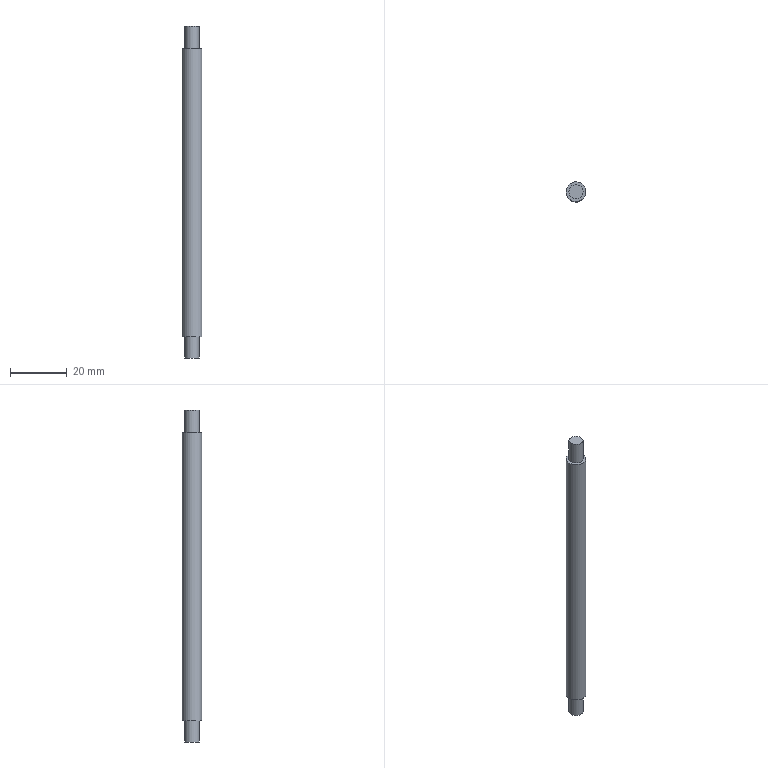Component | NX | COLUMN_4 | 1 solid | 7 faces | box 7 x 7 x 117.5 mm | volume 4230 mm3 | plane 4 | cylinder 3 | commonest cylinder face diameters 5 x2 7 x1
STEP:
#1=CARTESIAN_POINT('',(0.,0.,0.));
#2=DIRECTION('',(0.,0.,1.));
#3=DIRECTION('',(1.,0.,0.));
#4=AXIS2_PLACEMENT_3D('',#1,#2,#3);
#5=CARTESIAN_POINT('',(-21.585,4.647,11.));
#6=VERTEX_POINT('',#5);
#7=CARTESIAN_POINT('',(-24.,4.,11.));
#8=DIRECTION('',(0.,0.,1.));
#9=DIRECTION('',(0.9659,0.2588,0.));
#10=AXIS2_PLACEMENT_3D('',#7,#8,#9);
#11=CIRCLE('',#10,2.5);
#12=CARTESIAN_POINT('',(-24.,4.,11.));
#13=DIRECTION('',(0.,0.,-1.));
#14=DIRECTION('',(-0.9659,-0.2588,0.));
#15=AXIS2_PLACEMENT_3D('',#12,#13,#14);
#16=PLANE('',#15);
#17=CARTESIAN_POINT('',(-2.5,-0.));
#18=CARTESIAN_POINT('',(-2.5,4.33));
#19=CARTESIAN_POINT('',(1.25,2.165));
#20=CARTESIAN_POINT('',(5.,0.));
#21=CARTESIAN_POINT('',(1.25,-2.165));
#22=CARTESIAN_POINT('',(-2.5,-4.33));
#23=CARTESIAN_POINT('',(-2.5,-0.));
#24=(BOUNDED_CURVE()B_SPLINE_CURVE(2,(#17,#18,#19,#20,#21,#22,#23),.UNSPECIFIED.,.T.,.F.)B_SPLINE_CURVE_WITH_KNOTS((1,2,2,2,2,1),(-2.094,0.,2.094,4.189,6.283,8.378),.UNSPECIFIED.)CURVE()GEOMETRIC_REPRESENTATION_ITEM()RATIONAL_B_SPLINE_CURVE((1.,0.5,1.,0.5,1.,0.5,1.))REPRESENTATION_ITEM(''));
#25=(GEOMETRIC_REPRESENTATION_CONTEXT(2)PARAMETRIC_REPRESENTATION_CONTEXT()REPRESENTATION_CONTEXT('',''));
#26=DEFINITIONAL_REPRESENTATION('',(#24),#25);
#27=PCURVE('',#16,#26);
#28=CARTESIAN_POINT('',(-24.,4.,11.));
#29=DIRECTION('',(0.,0.,1.));
#30=DIRECTION('',(0.9659,0.2588,0.));
#31=AXIS2_PLACEMENT_3D('',#28,#29,#30);
#32=CYLINDRICAL_SURFACE('',#31,2.5);
#33=CARTESIAN_POINT('',(0.,0.));
#34=DIRECTION('',(1.,0.));
#35=VECTOR('',#34,1.);
#36=LINE('',#33,#35);
#37=(GEOMETRIC_REPRESENTATION_CONTEXT(2)PARAMETRIC_REPRESENTATION_CONTEXT()REPRESENTATION_CONTEXT('',''));
#38=DEFINITIONAL_REPRESENTATION('',(#36),#37);
#39=PCURVE('',#32,#38);
#40=SURFACE_CURVE('',#11,(#27,#39),.PCURVE_S1.);
#41=EDGE_CURVE('',#6,#6,#40,.T.);
#42=ORIENTED_EDGE('',*,*,#41,.F.);
#43=EDGE_LOOP('',(#42));
#44=FACE_BOUND('',#43,.T.);
#45=ADVANCED_FACE('',(#44),#16,.T.);
#46=CARTESIAN_POINT('',(-21.585,4.647,18.5));
#47=VERTEX_POINT('',#46);
#48=CARTESIAN_POINT('',(-24.,4.,18.5));
#49=DIRECTION('',(0.,0.,-1.));
#50=DIRECTION('',(0.9659,0.2588,0.));
#51=AXIS2_PLACEMENT_3D('',#48,#49,#50);
#52=CIRCLE('',#51,2.5);
#53=CARTESIAN_POINT('',(6.283,7.5));
#54=DIRECTION('',(-1.,0.));
#55=VECTOR('',#54,1.);
#56=LINE('',#53,#55);
#57=(GEOMETRIC_REPRESENTATION_CONTEXT(2)PARAMETRIC_REPRESENTATION_CONTEXT()REPRESENTATION_CONTEXT('',''));
#58=DEFINITIONAL_REPRESENTATION('',(#56),#57);
#59=PCURVE('',#32,#58);
#60=CARTESIAN_POINT('',(-24.,4.,18.5));
#61=DIRECTION('',(0.,0.,-1.));
#62=DIRECTION('',(-0.9659,-0.2588,0.));
#63=AXIS2_PLACEMENT_3D('',#60,#61,#62);
#64=PLANE('',#63);
#65=CARTESIAN_POINT('',(0.,0.));
#66=DIRECTION('',(-1.,-0.));
#67=AXIS2_PLACEMENT_2D('',#65,#66);
#68=CIRCLE('',#67,2.5);
#69=(GEOMETRIC_REPRESENTATION_CONTEXT(2)PARAMETRIC_REPRESENTATION_CONTEXT()REPRESENTATION_CONTEXT('',''));
#70=DEFINITIONAL_REPRESENTATION('',(#68),#69);
#71=PCURVE('',#64,#70);
#72=SURFACE_CURVE('',#52,(#59,#71),.PCURVE_S1.);
#73=EDGE_CURVE('',#47,#47,#72,.T.);
#74=ORIENTED_EDGE('',*,*,#73,.T.);
#75=CARTESIAN_POINT('',(-21.585,4.647,11.));
#76=CARTESIAN_POINT('',(-21.585,4.647,18.5));
#77=B_SPLINE_CURVE_WITH_KNOTS('',1,(#75,#76),.UNSPECIFIED.,.F.,.F.,(2,2),(0.,7.5),.PIECEWISE_BEZIER_KNOTS.);
#78=CARTESIAN_POINT('',(0.,0.));
#79=DIRECTION('',(0.,1.));
#80=VECTOR('',#79,1.);
#81=LINE('',#78,#80);
#82=(GEOMETRIC_REPRESENTATION_CONTEXT(2)PARAMETRIC_REPRESENTATION_CONTEXT()REPRESENTATION_CONTEXT('',''));
#83=DEFINITIONAL_REPRESENTATION('',(#81),#82);
#84=PCURVE('',#32,#83);
#85=CARTESIAN_POINT('',(6.283,0.));
#86=DIRECTION('',(0.,1.));
#87=VECTOR('',#86,1.);
#88=LINE('',#85,#87);
#89=(GEOMETRIC_REPRESENTATION_CONTEXT(2)PARAMETRIC_REPRESENTATION_CONTEXT()REPRESENTATION_CONTEXT('',''));
#90=DEFINITIONAL_REPRESENTATION('',(#88),#89);
#91=PCURVE('',#32,#90);
#92=SEAM_CURVE('',#77,(#84,#91),.PCURVE_S1.);
#93=EDGE_CURVE('',#6,#47,#92,.T.);
#94=ORIENTED_EDGE('',*,*,#93,.F.);
#95=ORIENTED_EDGE('',*,*,#41,.T.);
#96=ORIENTED_EDGE('',*,*,#93,.T.);
#97=EDGE_LOOP('',(#74,#94,#95,#96));
#98=FACE_BOUND('',#97,.T.);
#99=ADVANCED_FACE('',(#98),#32,.T.);
#100=CARTESIAN_POINT('',(-21.585,4.647,120.5));
#101=VERTEX_POINT('',#100);
#102=CARTESIAN_POINT('',(-24.,4.,120.5));
#103=DIRECTION('',(0.,0.,1.));
#104=DIRECTION('',(0.9659,0.2588,0.));
#105=AXIS2_PLACEMENT_3D('',#102,#103,#104);
#106=CIRCLE('',#105,2.5);
#107=CARTESIAN_POINT('',(-24.,4.,120.5));
#108=DIRECTION('',(0.,0.,1.));
#109=DIRECTION('',(0.9659,0.2588,0.));
#110=AXIS2_PLACEMENT_3D('',#107,#108,#109);
#111=PLANE('',#110);
#112=CARTESIAN_POINT('',(0.,0.));
#113=DIRECTION('',(1.,-0.));
#114=AXIS2_PLACEMENT_2D('',#112,#113);
#115=CIRCLE('',#114,2.5);
#116=(GEOMETRIC_REPRESENTATION_CONTEXT(2)PARAMETRIC_REPRESENTATION_CONTEXT()REPRESENTATION_CONTEXT('',''));
#117=DEFINITIONAL_REPRESENTATION('',(#115),#116);
#118=PCURVE('',#111,#117);
#119=CARTESIAN_POINT('',(-24.,4.,120.5));
#120=DIRECTION('',(0.,0.,1.));
#121=DIRECTION('',(0.9659,0.2588,0.));
#122=AXIS2_PLACEMENT_3D('',#119,#120,#121);
#123=CYLINDRICAL_SURFACE('',#122,2.5);
#124=CARTESIAN_POINT('',(0.,0.));
#125=DIRECTION('',(1.,0.));
#126=VECTOR('',#125,1.);
#127=LINE('',#124,#126);
#128=(GEOMETRIC_REPRESENTATION_CONTEXT(2)PARAMETRIC_REPRESENTATION_CONTEXT()REPRESENTATION_CONTEXT('',''));
#129=DEFINITIONAL_REPRESENTATION('',(#127),#128);
#130=PCURVE('',#123,#129);
#131=SURFACE_CURVE('',#106,(#118,#130),.PCURVE_S1.);
#132=EDGE_CURVE('',#101,#101,#131,.T.);
#133=ORIENTED_EDGE('',*,*,#132,.F.);
#134=EDGE_LOOP('',(#133));
#135=FACE_BOUND('',#134,.T.);
#136=CARTESIAN_POINT('',(-20.619,4.906,120.5));
#137=VERTEX_POINT('',#136);
#138=CARTESIAN_POINT('',(-24.,4.,120.5));
#139=DIRECTION('',(0.,0.,1.));
#140=DIRECTION('',(0.9659,0.2588,0.));
#141=AXIS2_PLACEMENT_3D('',#138,#139,#140);
#142=CIRCLE('',#141,3.5);
#143=CARTESIAN_POINT('',(0.,0.));
#144=DIRECTION('',(1.,0.));
#145=AXIS2_PLACEMENT_2D('',#143,#144);
#146=CIRCLE('',#145,3.5);
#147=(GEOMETRIC_REPRESENTATION_CONTEXT(2)PARAMETRIC_REPRESENTATION_CONTEXT()REPRESENTATION_CONTEXT('',''));
#148=DEFINITIONAL_REPRESENTATION('',(#146),#147);
#149=PCURVE('',#111,#148);
#150=CARTESIAN_POINT('',(-24.,4.,18.5));
#151=DIRECTION('',(0.,0.,1.));
#152=DIRECTION('',(0.9659,0.2588,0.));
#153=AXIS2_PLACEMENT_3D('',#150,#151,#152);
#154=CYLINDRICAL_SURFACE('',#153,3.5);
#155=CARTESIAN_POINT('',(0.,102.));
#156=DIRECTION('',(1.,0.));
#157=VECTOR('',#156,1.);
#158=LINE('',#155,#157);
#159=(GEOMETRIC_REPRESENTATION_CONTEXT(2)PARAMETRIC_REPRESENTATION_CONTEXT()REPRESENTATION_CONTEXT('',''));
#160=DEFINITIONAL_REPRESENTATION('',(#158),#159);
#161=PCURVE('',#154,#160);
#162=SURFACE_CURVE('',#142,(#149,#161),.PCURVE_S1.);
#163=EDGE_CURVE('',#137,#137,#162,.T.);
#164=ORIENTED_EDGE('',*,*,#163,.T.);
#165=EDGE_LOOP('',(#164));
#166=FACE_BOUND('',#165,.T.);
#167=ADVANCED_FACE('',(#135,#166),#111,.T.);
#168=ORIENTED_EDGE('',*,*,#73,.F.);
#169=EDGE_LOOP('',(#168));
#170=FACE_BOUND('',#169,.T.);
#171=CARTESIAN_POINT('',(-20.619,4.906,18.5));
#172=VERTEX_POINT('',#171);
#173=CARTESIAN_POINT('',(-24.,4.,18.5));
#174=DIRECTION('',(0.,0.,1.));
#175=DIRECTION('',(0.9659,0.2588,0.));
#176=AXIS2_PLACEMENT_3D('',#173,#174,#175);
#177=CIRCLE('',#176,3.5);
#178=CARTESIAN_POINT('',(-3.5,0.));
#179=CARTESIAN_POINT('',(-3.5,6.062));
#180=CARTESIAN_POINT('',(1.75,3.031));
#181=CARTESIAN_POINT('',(7.,0.));
#182=CARTESIAN_POINT('',(1.75,-3.031));
#183=CARTESIAN_POINT('',(-3.5,-6.062));
#184=CARTESIAN_POINT('',(-3.5,0.));
#185=(BOUNDED_CURVE()B_SPLINE_CURVE(2,(#178,#179,#180,#181,#182,#183,#184),.UNSPECIFIED.,.T.,.F.)B_SPLINE_CURVE_WITH_KNOTS((1,2,2,2,2,1),(-2.094,0.,2.094,4.189,6.283,8.378),.UNSPECIFIED.)CURVE()GEOMETRIC_REPRESENTATION_ITEM()RATIONAL_B_SPLINE_CURVE((1.,0.5,1.,0.5,1.,0.5,1.))REPRESENTATION_ITEM(''));
#186=(GEOMETRIC_REPRESENTATION_CONTEXT(2)PARAMETRIC_REPRESENTATION_CONTEXT()REPRESENTATION_CONTEXT('',''));
#187=DEFINITIONAL_REPRESENTATION('',(#185),#186);
#188=PCURVE('',#64,#187);
#189=CARTESIAN_POINT('',(0.,0.));
#190=DIRECTION('',(1.,0.));
#191=VECTOR('',#190,1.);
#192=LINE('',#189,#191);
#193=(GEOMETRIC_REPRESENTATION_CONTEXT(2)PARAMETRIC_REPRESENTATION_CONTEXT()REPRESENTATION_CONTEXT('',''));
#194=DEFINITIONAL_REPRESENTATION('',(#192),#193);
#195=PCURVE('',#154,#194);
#196=SURFACE_CURVE('',#177,(#188,#195),.PCURVE_S1.);
#197=EDGE_CURVE('',#172,#172,#196,.T.);
#198=ORIENTED_EDGE('',*,*,#197,.F.);
#199=EDGE_LOOP('',(#198));
#200=FACE_BOUND('',#199,.T.);
#201=ADVANCED_FACE('',(#170,#200),#64,.T.);
#202=ORIENTED_EDGE('',*,*,#163,.F.);
#203=CARTESIAN_POINT('',(-20.619,4.906,18.5));
#204=CARTESIAN_POINT('',(-20.619,4.906,120.5));
#205=B_SPLINE_CURVE_WITH_KNOTS('',1,(#203,#204),.UNSPECIFIED.,.F.,.F.,(2,2),(0.,102.),.PIECEWISE_BEZIER_KNOTS.);
#206=CARTESIAN_POINT('',(0.,0.));
#207=DIRECTION('',(0.,1.));
#208=VECTOR('',#207,1.);
#209=LINE('',#206,#208);
#210=(GEOMETRIC_REPRESENTATION_CONTEXT(2)PARAMETRIC_REPRESENTATION_CONTEXT()REPRESENTATION_CONTEXT('',''));
#211=DEFINITIONAL_REPRESENTATION('',(#209),#210);
#212=PCURVE('',#154,#211);
#213=CARTESIAN_POINT('',(6.283,0.));
#214=DIRECTION('',(0.,1.));
#215=VECTOR('',#214,1.);
#216=LINE('',#213,#215);
#217=(GEOMETRIC_REPRESENTATION_CONTEXT(2)PARAMETRIC_REPRESENTATION_CONTEXT()REPRESENTATION_CONTEXT('',''));
#218=DEFINITIONAL_REPRESENTATION('',(#216),#217);
#219=PCURVE('',#154,#218);
#220=SEAM_CURVE('',#205,(#212,#219),.PCURVE_S1.);
#221=EDGE_CURVE('',#172,#137,#220,.T.);
#222=ORIENTED_EDGE('',*,*,#221,.F.);
#223=ORIENTED_EDGE('',*,*,#197,.T.);
#224=ORIENTED_EDGE('',*,*,#221,.T.);
#225=EDGE_LOOP('',(#202,#222,#223,#224));
#226=FACE_BOUND('',#225,.T.);
#227=ADVANCED_FACE('',(#226),#154,.T.);
#228=CARTESIAN_POINT('',(-21.585,4.647,128.5));
#229=VERTEX_POINT('',#228);
#230=CARTESIAN_POINT('',(-24.,4.,128.5));
#231=DIRECTION('',(0.,0.,1.));
#232=DIRECTION('',(0.9659,0.2588,0.));
#233=AXIS2_PLACEMENT_3D('',#230,#231,#232);
#234=CIRCLE('',#233,2.5);
#235=CARTESIAN_POINT('',(-24.,4.,128.5));
#236=DIRECTION('',(0.,0.,1.));
#237=DIRECTION('',(0.9659,0.2588,0.));
#238=AXIS2_PLACEMENT_3D('',#235,#236,#237);
#239=PLANE('',#238);
#240=CARTESIAN_POINT('',(0.,0.));
#241=DIRECTION('',(1.,-0.));
#242=AXIS2_PLACEMENT_2D('',#240,#241);
#243=CIRCLE('',#242,2.5);
#244=(GEOMETRIC_REPRESENTATION_CONTEXT(2)PARAMETRIC_REPRESENTATION_CONTEXT()REPRESENTATION_CONTEXT('',''));
#245=DEFINITIONAL_REPRESENTATION('',(#243),#244);
#246=PCURVE('',#239,#245);
#247=CARTESIAN_POINT('',(0.,8.));
#248=DIRECTION('',(1.,0.));
#249=VECTOR('',#248,1.);
#250=LINE('',#247,#249);
#251=(GEOMETRIC_REPRESENTATION_CONTEXT(2)PARAMETRIC_REPRESENTATION_CONTEXT()REPRESENTATION_CONTEXT('',''));
#252=DEFINITIONAL_REPRESENTATION('',(#250),#251);
#253=PCURVE('',#123,#252);
#254=SURFACE_CURVE('',#234,(#246,#253),.PCURVE_S1.);
#255=EDGE_CURVE('',#229,#229,#254,.T.);
#256=ORIENTED_EDGE('',*,*,#255,.T.);
#257=EDGE_LOOP('',(#256));
#258=FACE_BOUND('',#257,.T.);
#259=ADVANCED_FACE('',(#258),#239,.T.);
#260=ORIENTED_EDGE('',*,*,#255,.F.);
#261=CARTESIAN_POINT('',(-21.585,4.647,120.5));
#262=CARTESIAN_POINT('',(-21.585,4.647,128.5));
#263=B_SPLINE_CURVE_WITH_KNOTS('',1,(#261,#262),.UNSPECIFIED.,.F.,.F.,(2,2),(0.,8.),.PIECEWISE_BEZIER_KNOTS.);
#264=CARTESIAN_POINT('',(0.,0.));
#265=DIRECTION('',(0.,1.));
#266=VECTOR('',#265,1.);
#267=LINE('',#264,#266);
#268=(GEOMETRIC_REPRESENTATION_CONTEXT(2)PARAMETRIC_REPRESENTATION_CONTEXT()REPRESENTATION_CONTEXT('',''));
#269=DEFINITIONAL_REPRESENTATION('',(#267),#268);
#270=PCURVE('',#123,#269);
#271=CARTESIAN_POINT('',(6.283,0.));
#272=DIRECTION('',(0.,1.));
#273=VECTOR('',#272,1.);
#274=LINE('',#271,#273);
#275=(GEOMETRIC_REPRESENTATION_CONTEXT(2)PARAMETRIC_REPRESENTATION_CONTEXT()REPRESENTATION_CONTEXT('',''));
#276=DEFINITIONAL_REPRESENTATION('',(#274),#275);
#277=PCURVE('',#123,#276);
#278=SEAM_CURVE('',#263,(#270,#277),.PCURVE_S1.);
#279=EDGE_CURVE('',#101,#229,#278,.T.);
#280=ORIENTED_EDGE('',*,*,#279,.F.);
#281=ORIENTED_EDGE('',*,*,#132,.T.);
#282=ORIENTED_EDGE('',*,*,#279,.T.);
#283=EDGE_LOOP('',(#260,#280,#281,#282));
#284=FACE_BOUND('',#283,.T.);
#285=ADVANCED_FACE('',(#284),#123,.T.);
#286=CLOSED_SHELL('',(#45,#99,#167,#201,#227,#259,#285));
#287=MANIFOLD_SOLID_BREP('',#286);
#288=(LENGTH_UNIT()NAMED_UNIT(*)SI_UNIT(.MILLI.,.METRE.));
#289=UNCERTAINTY_MEASURE_WITH_UNIT(LENGTH_MEASURE(0.00001),#288,'','');
#290=(NAMED_UNIT(*)PLANE_ANGLE_UNIT()SI_UNIT($,.RADIAN.));
#291=(NAMED_UNIT(*)SI_UNIT($,.STERADIAN.)SOLID_ANGLE_UNIT());
#292=(GEOMETRIC_REPRESENTATION_CONTEXT(3)GLOBAL_UNCERTAINTY_ASSIGNED_CONTEXT((#289))GLOBAL_UNIT_ASSIGNED_CONTEXT((#288,#290,#291))REPRESENTATION_CONTEXT('',''));
#293=ADVANCED_BREP_SHAPE_REPRESENTATION('',(#4,#287),#292);